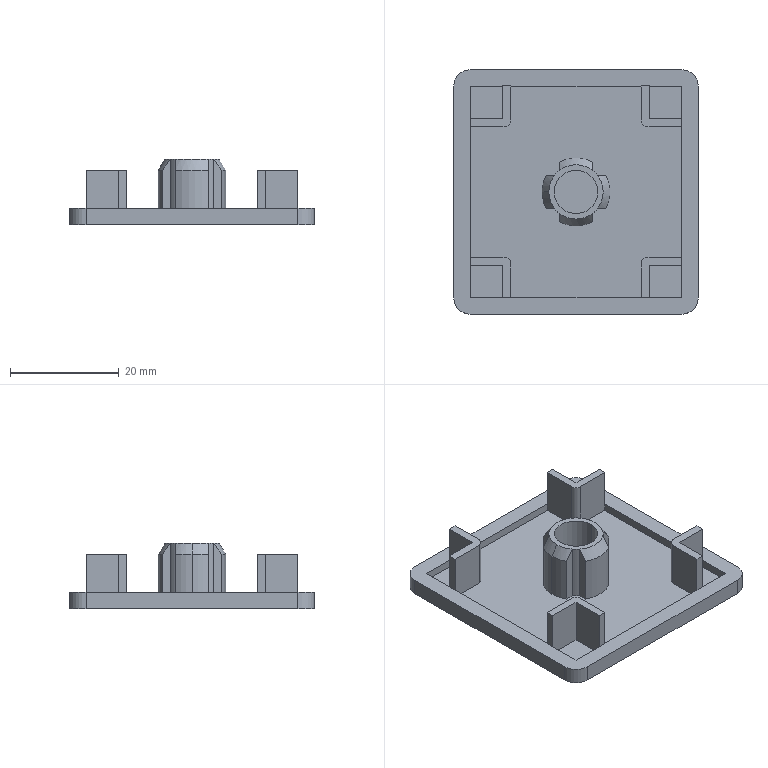Component | SolidWorks | HFC8_4545_B-2_HFC8_4545_Bc-1 | 1 solid | 85 faces | box 45 x 45 x 12 mm | volume 5045 mm3 | plane 61 | cylinder 19 | cone 5 | commonest cylinder face diameters 12.5 x5 6 x4 10 x4 2.5 x4 8 x2
build123d program:
from build123d import *

# Parameters (mm, degrees)
BOSS_EXTRUDE1_DEPTH      = 3
SKETCH2_W                = 39
SKETCH2_H                = 39
CUT_EXTRUDE1_DEPTH       = 1.5
BOSS_EXTRUDE2_DEPTH      = 8.5
BOSS_EXTRUDE3_DEPTH      = 8.5
BOSS_EXTRUDE4_DEPTH      = 8.5
BOSS_EXTRUDE5_DEPTH      = 8.5
SKETCH8_R                = 8
CUT_EXTRUDE2_DEPTH       = 12
PLUGCORNERRELIEF_R1_25_R = 1.25


with BuildPart() as part:
    # Sketch1 → Boss-Extrude1 (new body)
    with BuildSketch(Plane.XY):
        with BuildLine():
            Line((-22.5, 19.5), (-22.5, -19.5))
            ThreePointArc((-22.5, -19.5), (-21.621, -21.621), (-19.5, -22.5))
            Line((-19.5, -22.5), (19.5, -22.5))
            ThreePointArc((19.5, -22.5), (21.621, -21.621), (22.5, -19.5))
            Line((22.5, -19.5), (22.5, 19.5))
            ThreePointArc((22.5, 19.5), (21.621, 21.621), (19.5, 22.5))
            Line((19.5, 22.5), (-19.5, 22.5))
            ThreePointArc((-19.5, 22.5), (-21.621, 21.621), (-22.5, 19.5))
        make_face()
    extrude(amount=-BOSS_EXTRUDE1_DEPTH)

    # Sketch2 → Cut-Extrude1 (cut)
    with BuildSketch(Plane.XY):
        Rectangle(SKETCH2_W, SKETCH2_H)
    extrude(amount=-CUT_EXTRUDE1_DEPTH, mode=Mode.SUBTRACT)

    # Sketch3 → Boss-Extrude2 (add)
    with BuildSketch(Plane.XY.offset(-1.5)):
        Polygon((-19.5, 12), (-12, 12), (-12, 19.5), (-13.5, 19.5), (-13.5, 13.5), (-19.5, 13.5), align=None)
    extrude(amount=BOSS_EXTRUDE2_DEPTH)

    # Sketch4 → Boss-Extrude3 (add)
    with BuildSketch(Plane.XY.offset(-1.5)):
        Polygon((12, 19.5), (12, 12), (19.5, 12), (19.5, 13.5), (13.5, 13.5), (13.5, 19.5), align=None)
    extrude(amount=BOSS_EXTRUDE3_DEPTH)

    # Sketch5 → Boss-Extrude4 (add)
    with BuildSketch(Plane.XY.offset(-1.5)):
        Polygon((-19.5, -12), (-19.5, -13.5), (-13.5, -13.5), (-13.5, -19.5), (-12, -19.5), (-12, -12), align=None)
    extrude(amount=BOSS_EXTRUDE4_DEPTH)

    # Sketch6 → Boss-Extrude5 (add)
    with BuildSketch(Plane.XY.offset(-1.5)):
        Polygon((12, -19.5), (13.5, -19.5), (13.5, -13.5), (19.5, -13.5), (19.5, -12), (12, -12), align=None)
    extrude(amount=BOSS_EXTRUDE5_DEPTH)

    # Sketch7 → Revolve1 (revolve)
    with BuildSketch(Plane(origin=(0, 0, 0), x_dir=(1, 0, 0), z_dir=(0, 1, 0)), mode=Mode.PRIVATE) as revolve1_sk:
        Polygon((4, 1.5), (4, -9), (5, -9), (6.25, -7), (6.25, 1.5), align=None)
    revolve(revolve1_sk.sketch.rotate(Axis((0, 0, 9), (0, 0, -1)), 180), axis=Axis((0, 0, 9), (0, 0, -1)))

    # Sketch8 → Cut-Extrude2 (cut)
    with BuildSketch(Plane.XY.offset(-1.5)):
        Circle(SKETCH8_R)
        with BuildLine():
            Line((-5.483, -3), (-4, -3))
            ThreePointArc((-4, -3), (-3.536, -3.536), (-3, -4))
            Line((-3, -4), (-3, -5.483))
            ThreePointArc((-3, -5.483), (0, -6.25), (3, -5.483))
            Line((3, -5.483), (3, -4))
            ThreePointArc((3, -4), (3.536, -3.536), (4, -3))
            Line((4, -3), (5.483, -3))
            ThreePointArc((5.483, -3), (6.25, 0), (5.483, 3))
            Line((5.483, 3), (4, 3))
            ThreePointArc((4, 3), (3.536, 3.536), (3, 4))
            Line((3, 4), (3, 5.483))
            ThreePointArc((3, 5.483), (0, 6.25), (-3, 5.483))
            Line((-3, 5.483), (-3, 4))
            ThreePointArc((-3, 4), (-3.536, 3.536), (-4, 3))
            Line((-4, 3), (-5.483, 3))
            ThreePointArc((-5.483, 3), (-6.25, 0), (-5.483, -3))
        make_face(mode=Mode.SUBTRACT)
    extrude(amount=CUT_EXTRUDE2_DEPTH, mode=Mode.SUBTRACT)

    # PlugCornerRelief_R1.25
    plugcornerrelief_r1_25_edges = [part.edges().sort_by_distance(p)[0] for p in [
        (12, -12, 2.75),
        (-12, 12, 2.75),
        (12, 12, 2.75),
        (-12, -12, 2.75),
    ]]
    fillet(plugcornerrelief_r1_25_edges, radius=PLUGCORNERRELIEF_R1_25_R)


solid = part.part

# Placed as in the assembly
solid = solid.moved(Location((-65.506, 8.087, -2402.928), (0, 0, 0)))